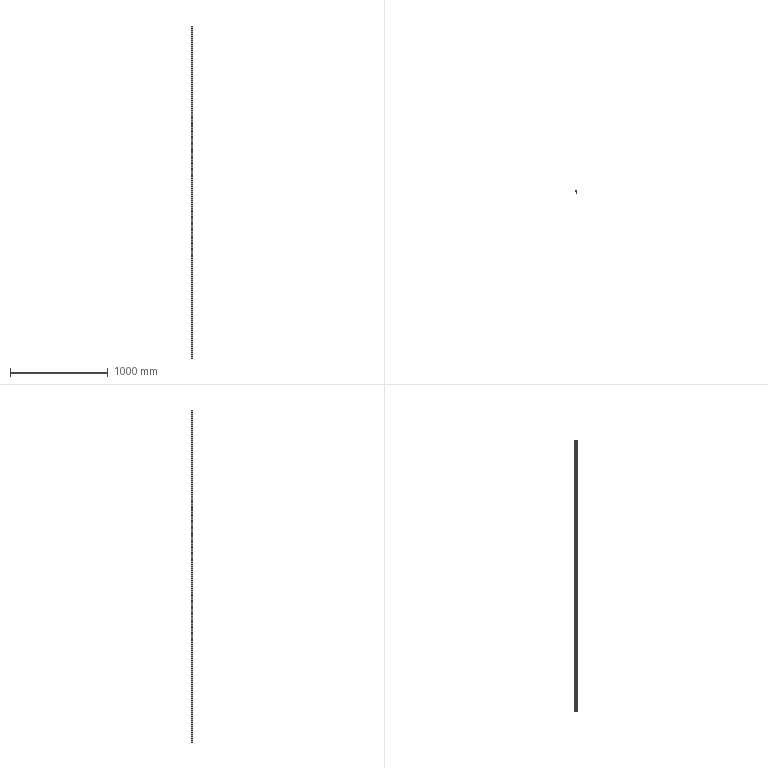Component | NX | RIB_STRIP_10 | 1 solid | 10 faces | box 14 x 15 x 3390 mm | volume 304388 mm3 | plane 10
STEP:
#1=CARTESIAN_POINT('',(0.,0.,0.));
#2=DIRECTION('',(0.,0.,1.));
#3=DIRECTION('',(1.,0.,0.));
#4=AXIS2_PLACEMENT_3D('',#1,#2,#3);
#5=CARTESIAN_POINT('',(6068.006,4310.094,-3362.));
#6=VERTEX_POINT('',#5);
#7=CARTESIAN_POINT('',(6068.006,4307.094,-3362.));
#8=VERTEX_POINT('',#7);
#9=CARTESIAN_POINT('',(6068.006,4310.094,-3362.));
#10=DIRECTION('',(0.,-1.,0.));
#11=VECTOR('',#10,1.);
#12=LINE('',#9,#11);
#13=CARTESIAN_POINT('',(6068.006,4310.094,28.));
#14=DIRECTION('',(1.,0.,0.));
#15=DIRECTION('',(0.,0.,-1.));
#16=AXIS2_PLACEMENT_3D('',#13,#14,#15);
#17=PLANE('',#16);
#18=CARTESIAN_POINT('',(3390.,0.));
#19=DIRECTION('',(0.,-1.));
#20=VECTOR('',#19,1.);
#21=LINE('',#18,#20);
#22=(GEOMETRIC_REPRESENTATION_CONTEXT(2)PARAMETRIC_REPRESENTATION_CONTEXT()REPRESENTATION_CONTEXT('',''));
#23=DEFINITIONAL_REPRESENTATION('',(#21),#22);
#24=PCURVE('',#17,#23);
#25=CARTESIAN_POINT('',(6068.006,4310.094,-3362.));
#26=DIRECTION('',(0.,0.,1.));
#27=DIRECTION('',(1.,0.,0.));
#28=AXIS2_PLACEMENT_3D('',#25,#26,#27);
#29=PLANE('',#28);
#30=CARTESIAN_POINT('',(0.,0.));
#31=DIRECTION('',(0.,-1.));
#32=VECTOR('',#31,1.);
#33=LINE('',#30,#32);
#34=(GEOMETRIC_REPRESENTATION_CONTEXT(2)PARAMETRIC_REPRESENTATION_CONTEXT()REPRESENTATION_CONTEXT('',''));
#35=DEFINITIONAL_REPRESENTATION('',(#33),#34);
#36=PCURVE('',#29,#35);
#37=SURFACE_CURVE('',#12,(#24,#36),.PCURVE_S1.);
#38=EDGE_CURVE('',#6,#8,#37,.T.);
#39=ORIENTED_EDGE('',*,*,#38,.T.);
#40=CARTESIAN_POINT('',(6068.006,4307.094,28.));
#41=VERTEX_POINT('',#40);
#42=CARTESIAN_POINT('',(6068.006,4307.094,28.));
#43=DIRECTION('',(0.,0.,-1.));
#44=VECTOR('',#43,1.);
#45=LINE('',#42,#44);
#46=CARTESIAN_POINT('',(0.,-3.));
#47=DIRECTION('',(1.,0.));
#48=VECTOR('',#47,1.);
#49=LINE('',#46,#48);
#50=(GEOMETRIC_REPRESENTATION_CONTEXT(2)PARAMETRIC_REPRESENTATION_CONTEXT()REPRESENTATION_CONTEXT('',''));
#51=DEFINITIONAL_REPRESENTATION('',(#49),#50);
#52=PCURVE('',#17,#51);
#53=CARTESIAN_POINT('',(6068.006,4307.094,28.));
#54=DIRECTION('',(0.,1.,0.));
#55=DIRECTION('',(0.,0.,1.));
#56=AXIS2_PLACEMENT_3D('',#53,#54,#55);
#57=PLANE('',#56);
#58=CARTESIAN_POINT('',(0.,0.));
#59=DIRECTION('',(-1.,0.));
#60=VECTOR('',#59,1.);
#61=LINE('',#58,#60);
#62=(GEOMETRIC_REPRESENTATION_CONTEXT(2)PARAMETRIC_REPRESENTATION_CONTEXT()REPRESENTATION_CONTEXT('',''));
#63=DEFINITIONAL_REPRESENTATION('',(#61),#62);
#64=PCURVE('',#57,#63);
#65=SURFACE_CURVE('',#45,(#52,#64),.PCURVE_S1.);
#66=EDGE_CURVE('',#41,#8,#65,.T.);
#67=ORIENTED_EDGE('',*,*,#66,.F.);
#68=CARTESIAN_POINT('',(6068.006,4310.094,28.));
#69=VERTEX_POINT('',#68);
#70=CARTESIAN_POINT('',(6068.006,4310.094,28.));
#71=DIRECTION('',(0.,-1.,0.));
#72=VECTOR('',#71,1.);
#73=LINE('',#70,#72);
#74=CARTESIAN_POINT('',(0.,0.));
#75=DIRECTION('',(0.,-1.));
#76=VECTOR('',#75,1.);
#77=LINE('',#74,#76);
#78=(GEOMETRIC_REPRESENTATION_CONTEXT(2)PARAMETRIC_REPRESENTATION_CONTEXT()REPRESENTATION_CONTEXT('',''));
#79=DEFINITIONAL_REPRESENTATION('',(#77),#78);
#80=PCURVE('',#17,#79);
#81=CARTESIAN_POINT('',(6068.006,4310.094,28.));
#82=DIRECTION('',(0.,0.,1.));
#83=DIRECTION('',(1.,0.,0.));
#84=AXIS2_PLACEMENT_3D('',#81,#82,#83);
#85=PLANE('',#84);
#86=CARTESIAN_POINT('',(0.,0.));
#87=DIRECTION('',(0.,-1.));
#88=VECTOR('',#87,1.);
#89=LINE('',#86,#88);
#90=(GEOMETRIC_REPRESENTATION_CONTEXT(2)PARAMETRIC_REPRESENTATION_CONTEXT()REPRESENTATION_CONTEXT('',''));
#91=DEFINITIONAL_REPRESENTATION('',(#89),#90);
#92=PCURVE('',#85,#91);
#93=SURFACE_CURVE('',#73,(#80,#92),.PCURVE_S1.);
#94=EDGE_CURVE('',#69,#41,#93,.T.);
#95=ORIENTED_EDGE('',*,*,#94,.F.);
#96=CARTESIAN_POINT('',(6068.006,4310.094,28.));
#97=DIRECTION('',(0.,0.,-1.));
#98=VECTOR('',#97,1.);
#99=LINE('',#96,#98);
#100=CARTESIAN_POINT('',(0.,0.));
#101=DIRECTION('',(1.,0.));
#102=VECTOR('',#101,1.);
#103=LINE('',#100,#102);
#104=(GEOMETRIC_REPRESENTATION_CONTEXT(2)PARAMETRIC_REPRESENTATION_CONTEXT()REPRESENTATION_CONTEXT('',''));
#105=DEFINITIONAL_REPRESENTATION('',(#103),#104);
#106=PCURVE('',#17,#105);
#107=CARTESIAN_POINT('',(6082.006,4310.094,28.));
#108=DIRECTION('',(0.,-1.,0.));
#109=DIRECTION('',(0.,0.,-1.));
#110=AXIS2_PLACEMENT_3D('',#107,#108,#109);
#111=PLANE('',#110);
#112=CARTESIAN_POINT('',(0.,-14.));
#113=DIRECTION('',(1.,0.));
#114=VECTOR('',#113,1.);
#115=LINE('',#112,#114);
#116=(GEOMETRIC_REPRESENTATION_CONTEXT(2)PARAMETRIC_REPRESENTATION_CONTEXT()REPRESENTATION_CONTEXT('',''));
#117=DEFINITIONAL_REPRESENTATION('',(#115),#116);
#118=PCURVE('',#111,#117);
#119=SURFACE_CURVE('',#99,(#106,#118),.PCURVE_S1.);
#120=EDGE_CURVE('',#69,#6,#119,.T.);
#121=ORIENTED_EDGE('',*,*,#120,.T.);
#122=EDGE_LOOP('',(#39,#67,#95,#121));
#123=FACE_BOUND('',#122,.T.);
#124=ADVANCED_FACE('',(#123),#17,.F.);
#125=CARTESIAN_POINT('',(6079.006,4307.094,-3362.));
#126=VERTEX_POINT('',#125);
#127=CARTESIAN_POINT('',(6068.006,4307.094,-3362.));
#128=DIRECTION('',(1.,0.,0.));
#129=VECTOR('',#128,1.);
#130=LINE('',#127,#129);
#131=CARTESIAN_POINT('',(-3390.,0.));
#132=DIRECTION('',(0.,1.));
#133=VECTOR('',#132,1.);
#134=LINE('',#131,#133);
#135=(GEOMETRIC_REPRESENTATION_CONTEXT(2)PARAMETRIC_REPRESENTATION_CONTEXT()REPRESENTATION_CONTEXT('',''));
#136=DEFINITIONAL_REPRESENTATION('',(#134),#135);
#137=PCURVE('',#57,#136);
#138=CARTESIAN_POINT('',(0.,-3.));
#139=DIRECTION('',(1.,0.));
#140=VECTOR('',#139,1.);
#141=LINE('',#138,#140);
#142=(GEOMETRIC_REPRESENTATION_CONTEXT(2)PARAMETRIC_REPRESENTATION_CONTEXT()REPRESENTATION_CONTEXT('',''));
#143=DEFINITIONAL_REPRESENTATION('',(#141),#142);
#144=PCURVE('',#29,#143);
#145=SURFACE_CURVE('',#130,(#137,#144),.PCURVE_S1.);
#146=EDGE_CURVE('',#8,#126,#145,.T.);
#147=ORIENTED_EDGE('',*,*,#146,.T.);
#148=CARTESIAN_POINT('',(6079.006,4307.094,28.));
#149=VERTEX_POINT('',#148);
#150=CARTESIAN_POINT('',(6079.006,4307.094,28.));
#151=DIRECTION('',(0.,0.,-1.));
#152=VECTOR('',#151,1.);
#153=LINE('',#150,#152);
#154=CARTESIAN_POINT('',(0.,11.));
#155=DIRECTION('',(-1.,0.));
#156=VECTOR('',#155,1.);
#157=LINE('',#154,#156);
#158=(GEOMETRIC_REPRESENTATION_CONTEXT(2)PARAMETRIC_REPRESENTATION_CONTEXT()REPRESENTATION_CONTEXT('',''));
#159=DEFINITIONAL_REPRESENTATION('',(#157),#158);
#160=PCURVE('',#57,#159);
#161=CARTESIAN_POINT('',(6079.006,4307.094,28.));
#162=DIRECTION('',(1.,0.,0.));
#163=DIRECTION('',(0.,0.,-1.));
#164=AXIS2_PLACEMENT_3D('',#161,#162,#163);
#165=PLANE('',#164);
#166=CARTESIAN_POINT('',(0.,0.));
#167=DIRECTION('',(1.,0.));
#168=VECTOR('',#167,1.);
#169=LINE('',#166,#168);
#170=(GEOMETRIC_REPRESENTATION_CONTEXT(2)PARAMETRIC_REPRESENTATION_CONTEXT()REPRESENTATION_CONTEXT('',''));
#171=DEFINITIONAL_REPRESENTATION('',(#169),#170);
#172=PCURVE('',#165,#171);
#173=SURFACE_CURVE('',#153,(#160,#172),.PCURVE_S1.);
#174=EDGE_CURVE('',#149,#126,#173,.T.);
#175=ORIENTED_EDGE('',*,*,#174,.F.);
#176=CARTESIAN_POINT('',(6068.006,4307.094,28.));
#177=DIRECTION('',(1.,0.,0.));
#178=VECTOR('',#177,1.);
#179=LINE('',#176,#178);
#180=CARTESIAN_POINT('',(0.,0.));
#181=DIRECTION('',(0.,1.));
#182=VECTOR('',#181,1.);
#183=LINE('',#180,#182);
#184=(GEOMETRIC_REPRESENTATION_CONTEXT(2)PARAMETRIC_REPRESENTATION_CONTEXT()REPRESENTATION_CONTEXT('',''));
#185=DEFINITIONAL_REPRESENTATION('',(#183),#184);
#186=PCURVE('',#57,#185);
#187=CARTESIAN_POINT('',(0.,-3.));
#188=DIRECTION('',(1.,0.));
#189=VECTOR('',#188,1.);
#190=LINE('',#187,#189);
#191=(GEOMETRIC_REPRESENTATION_CONTEXT(2)PARAMETRIC_REPRESENTATION_CONTEXT()REPRESENTATION_CONTEXT('',''));
#192=DEFINITIONAL_REPRESENTATION('',(#190),#191);
#193=PCURVE('',#85,#192);
#194=SURFACE_CURVE('',#179,(#186,#193),.PCURVE_S1.);
#195=EDGE_CURVE('',#41,#149,#194,.T.);
#196=ORIENTED_EDGE('',*,*,#195,.F.);
#197=ORIENTED_EDGE('',*,*,#66,.T.);
#198=EDGE_LOOP('',(#147,#175,#196,#197));
#199=FACE_BOUND('',#198,.T.);
#200=ADVANCED_FACE('',(#199),#57,.F.);
#201=CARTESIAN_POINT('',(6079.006,4298.042,-3362.));
#202=VERTEX_POINT('',#201);
#203=CARTESIAN_POINT('',(6079.006,4307.094,-3362.));
#204=DIRECTION('',(0.,-1.,0.));
#205=VECTOR('',#204,1.);
#206=LINE('',#203,#205);
#207=CARTESIAN_POINT('',(3390.,0.));
#208=DIRECTION('',(0.,-1.));
#209=VECTOR('',#208,1.);
#210=LINE('',#207,#209);
#211=(GEOMETRIC_REPRESENTATION_CONTEXT(2)PARAMETRIC_REPRESENTATION_CONTEXT()REPRESENTATION_CONTEXT('',''));
#212=DEFINITIONAL_REPRESENTATION('',(#210),#211);
#213=PCURVE('',#165,#212);
#214=CARTESIAN_POINT('',(11.,-3.));
#215=DIRECTION('',(0.,-1.));
#216=VECTOR('',#215,1.);
#217=LINE('',#214,#216);
#218=(GEOMETRIC_REPRESENTATION_CONTEXT(2)PARAMETRIC_REPRESENTATION_CONTEXT()REPRESENTATION_CONTEXT('',''));
#219=DEFINITIONAL_REPRESENTATION('',(#217),#218);
#220=PCURVE('',#29,#219);
#221=SURFACE_CURVE('',#206,(#213,#220),.PCURVE_S1.);
#222=EDGE_CURVE('',#126,#202,#221,.T.);
#223=ORIENTED_EDGE('',*,*,#222,.T.);
#224=CARTESIAN_POINT('',(6079.006,4298.042,28.));
#225=VERTEX_POINT('',#224);
#226=CARTESIAN_POINT('',(6079.006,4298.042,28.));
#227=DIRECTION('',(0.,0.,-1.));
#228=VECTOR('',#227,1.);
#229=LINE('',#226,#228);
#230=CARTESIAN_POINT('',(0.,-9.052));
#231=DIRECTION('',(1.,0.));
#232=VECTOR('',#231,1.);
#233=LINE('',#230,#232);
#234=(GEOMETRIC_REPRESENTATION_CONTEXT(2)PARAMETRIC_REPRESENTATION_CONTEXT()REPRESENTATION_CONTEXT('',''));
#235=DEFINITIONAL_REPRESENTATION('',(#233),#234);
#236=PCURVE('',#165,#235);
#237=CARTESIAN_POINT('',(6079.006,4298.042,28.));
#238=DIRECTION('',(0.,-1.,0.));
#239=DIRECTION('',(0.,0.,-1.));
#240=AXIS2_PLACEMENT_3D('',#237,#238,#239);
#241=PLANE('',#240);
#242=CARTESIAN_POINT('',(0.,0.));
#243=DIRECTION('',(1.,0.));
#244=VECTOR('',#243,1.);
#245=LINE('',#242,#244);
#246=(GEOMETRIC_REPRESENTATION_CONTEXT(2)PARAMETRIC_REPRESENTATION_CONTEXT()REPRESENTATION_CONTEXT('',''));
#247=DEFINITIONAL_REPRESENTATION('',(#245),#246);
#248=PCURVE('',#241,#247);
#249=SURFACE_CURVE('',#229,(#236,#248),.PCURVE_S1.);
#250=EDGE_CURVE('',#225,#202,#249,.T.);
#251=ORIENTED_EDGE('',*,*,#250,.F.);
#252=CARTESIAN_POINT('',(6079.006,4307.094,28.));
#253=DIRECTION('',(0.,-1.,0.));
#254=VECTOR('',#253,1.);
#255=LINE('',#252,#254);
#256=CARTESIAN_POINT('',(0.,0.));
#257=DIRECTION('',(0.,-1.));
#258=VECTOR('',#257,1.);
#259=LINE('',#256,#258);
#260=(GEOMETRIC_REPRESENTATION_CONTEXT(2)PARAMETRIC_REPRESENTATION_CONTEXT()REPRESENTATION_CONTEXT('',''));
#261=DEFINITIONAL_REPRESENTATION('',(#259),#260);
#262=PCURVE('',#165,#261);
#263=CARTESIAN_POINT('',(11.,-3.));
#264=DIRECTION('',(0.,-1.));
#265=VECTOR('',#264,1.);
#266=LINE('',#263,#265);
#267=(GEOMETRIC_REPRESENTATION_CONTEXT(2)PARAMETRIC_REPRESENTATION_CONTEXT()REPRESENTATION_CONTEXT('',''));
#268=DEFINITIONAL_REPRESENTATION('',(#266),#267);
#269=PCURVE('',#85,#268);
#270=SURFACE_CURVE('',#255,(#262,#269),.PCURVE_S1.);
#271=EDGE_CURVE('',#149,#225,#270,.T.);
#272=ORIENTED_EDGE('',*,*,#271,.F.);
#273=ORIENTED_EDGE('',*,*,#174,.T.);
#274=EDGE_LOOP('',(#223,#251,#272,#273));
#275=FACE_BOUND('',#274,.T.);
#276=ADVANCED_FACE('',(#275),#165,.F.);
#277=CARTESIAN_POINT('',(6075.006,4298.042,-3362.));
#278=VERTEX_POINT('',#277);
#279=CARTESIAN_POINT('',(6079.006,4298.042,-3362.));
#280=DIRECTION('',(-1.,0.,0.));
#281=VECTOR('',#280,1.);
#282=LINE('',#279,#281);
#283=CARTESIAN_POINT('',(3390.,0.));
#284=DIRECTION('',(0.,-1.));
#285=VECTOR('',#284,1.);
#286=LINE('',#283,#285);
#287=(GEOMETRIC_REPRESENTATION_CONTEXT(2)PARAMETRIC_REPRESENTATION_CONTEXT()REPRESENTATION_CONTEXT('',''));
#288=DEFINITIONAL_REPRESENTATION('',(#286),#287);
#289=PCURVE('',#241,#288);
#290=CARTESIAN_POINT('',(11.,-12.052));
#291=DIRECTION('',(-1.,0.));
#292=VECTOR('',#291,1.);
#293=LINE('',#290,#292);
#294=(GEOMETRIC_REPRESENTATION_CONTEXT(2)PARAMETRIC_REPRESENTATION_CONTEXT()REPRESENTATION_CONTEXT('',''));
#295=DEFINITIONAL_REPRESENTATION('',(#293),#294);
#296=PCURVE('',#29,#295);
#297=SURFACE_CURVE('',#282,(#289,#296),.PCURVE_S1.);
#298=EDGE_CURVE('',#202,#278,#297,.T.);
#299=ORIENTED_EDGE('',*,*,#298,.T.);
#300=CARTESIAN_POINT('',(6075.006,4298.042,28.));
#301=VERTEX_POINT('',#300);
#302=CARTESIAN_POINT('',(6075.006,4298.042,28.));
#303=DIRECTION('',(0.,0.,-1.));
#304=VECTOR('',#303,1.);
#305=LINE('',#302,#304);
#306=CARTESIAN_POINT('',(0.,-4.));
#307=DIRECTION('',(1.,0.));
#308=VECTOR('',#307,1.);
#309=LINE('',#306,#308);
#310=(GEOMETRIC_REPRESENTATION_CONTEXT(2)PARAMETRIC_REPRESENTATION_CONTEXT()REPRESENTATION_CONTEXT('',''));
#311=DEFINITIONAL_REPRESENTATION('',(#309),#310);
#312=PCURVE('',#241,#311);
#313=CARTESIAN_POINT('',(6075.006,4298.042,28.));
#314=DIRECTION('',(1.,0.,0.));
#315=DIRECTION('',(0.,0.,-1.));
#316=AXIS2_PLACEMENT_3D('',#313,#314,#315);
#317=PLANE('',#316);
#318=CARTESIAN_POINT('',(0.,0.));
#319=DIRECTION('',(1.,0.));
#320=VECTOR('',#319,1.);
#321=LINE('',#318,#320);
#322=(GEOMETRIC_REPRESENTATION_CONTEXT(2)PARAMETRIC_REPRESENTATION_CONTEXT()REPRESENTATION_CONTEXT('',''));
#323=DEFINITIONAL_REPRESENTATION('',(#321),#322);
#324=PCURVE('',#317,#323);
#325=SURFACE_CURVE('',#305,(#312,#324),.PCURVE_S1.);
#326=EDGE_CURVE('',#301,#278,#325,.T.);
#327=ORIENTED_EDGE('',*,*,#326,.F.);
#328=CARTESIAN_POINT('',(6079.006,4298.042,28.));
#329=DIRECTION('',(-1.,0.,0.));
#330=VECTOR('',#329,1.);
#331=LINE('',#328,#330);
#332=CARTESIAN_POINT('',(0.,0.));
#333=DIRECTION('',(0.,-1.));
#334=VECTOR('',#333,1.);
#335=LINE('',#332,#334);
#336=(GEOMETRIC_REPRESENTATION_CONTEXT(2)PARAMETRIC_REPRESENTATION_CONTEXT()REPRESENTATION_CONTEXT('',''));
#337=DEFINITIONAL_REPRESENTATION('',(#335),#336);
#338=PCURVE('',#241,#337);
#339=CARTESIAN_POINT('',(11.,-12.052));
#340=DIRECTION('',(-1.,0.));
#341=VECTOR('',#340,1.);
#342=LINE('',#339,#341);
#343=(GEOMETRIC_REPRESENTATION_CONTEXT(2)PARAMETRIC_REPRESENTATION_CONTEXT()REPRESENTATION_CONTEXT('',''));
#344=DEFINITIONAL_REPRESENTATION('',(#342),#343);
#345=PCURVE('',#85,#344);
#346=SURFACE_CURVE('',#331,(#338,#345),.PCURVE_S1.);
#347=EDGE_CURVE('',#225,#301,#346,.T.);
#348=ORIENTED_EDGE('',*,*,#347,.F.);
#349=ORIENTED_EDGE('',*,*,#250,.T.);
#350=EDGE_LOOP('',(#299,#327,#348,#349));
#351=FACE_BOUND('',#350,.T.);
#352=ADVANCED_FACE('',(#351),#241,.F.);
#353=CARTESIAN_POINT('',(6075.006,4295.094,-3362.));
#354=VERTEX_POINT('',#353);
#355=CARTESIAN_POINT('',(6075.006,4298.042,-3362.));
#356=DIRECTION('',(0.,-1.,0.));
#357=VECTOR('',#356,1.);
#358=LINE('',#355,#357);
#359=CARTESIAN_POINT('',(3390.,0.));
#360=DIRECTION('',(0.,-1.));
#361=VECTOR('',#360,1.);
#362=LINE('',#359,#361);
#363=(GEOMETRIC_REPRESENTATION_CONTEXT(2)PARAMETRIC_REPRESENTATION_CONTEXT()REPRESENTATION_CONTEXT('',''));
#364=DEFINITIONAL_REPRESENTATION('',(#362),#363);
#365=PCURVE('',#317,#364);
#366=CARTESIAN_POINT('',(7.,-12.052));
#367=DIRECTION('',(0.,-1.));
#368=VECTOR('',#367,1.);
#369=LINE('',#366,#368);
#370=(GEOMETRIC_REPRESENTATION_CONTEXT(2)PARAMETRIC_REPRESENTATION_CONTEXT()REPRESENTATION_CONTEXT('',''));
#371=DEFINITIONAL_REPRESENTATION('',(#369),#370);
#372=PCURVE('',#29,#371);
#373=SURFACE_CURVE('',#358,(#365,#372),.PCURVE_S1.);
#374=EDGE_CURVE('',#278,#354,#373,.T.);
#375=ORIENTED_EDGE('',*,*,#374,.T.);
#376=CARTESIAN_POINT('',(6075.006,4295.094,28.));
#377=VERTEX_POINT('',#376);
#378=CARTESIAN_POINT('',(6075.006,4295.094,28.));
#379=DIRECTION('',(0.,0.,-1.));
#380=VECTOR('',#379,1.);
#381=LINE('',#378,#380);
#382=CARTESIAN_POINT('',(0.,-2.948));
#383=DIRECTION('',(1.,0.));
#384=VECTOR('',#383,1.);
#385=LINE('',#382,#384);
#386=(GEOMETRIC_REPRESENTATION_CONTEXT(2)PARAMETRIC_REPRESENTATION_CONTEXT()REPRESENTATION_CONTEXT('',''));
#387=DEFINITIONAL_REPRESENTATION('',(#385),#386);
#388=PCURVE('',#317,#387);
#389=CARTESIAN_POINT('',(6075.006,4295.094,28.));
#390=DIRECTION('',(0.,1.,0.));
#391=DIRECTION('',(0.,0.,1.));
#392=AXIS2_PLACEMENT_3D('',#389,#390,#391);
#393=PLANE('',#392);
#394=CARTESIAN_POINT('',(0.,0.));
#395=DIRECTION('',(-1.,0.));
#396=VECTOR('',#395,1.);
#397=LINE('',#394,#396);
#398=(GEOMETRIC_REPRESENTATION_CONTEXT(2)PARAMETRIC_REPRESENTATION_CONTEXT()REPRESENTATION_CONTEXT('',''));
#399=DEFINITIONAL_REPRESENTATION('',(#397),#398);
#400=PCURVE('',#393,#399);
#401=SURFACE_CURVE('',#381,(#388,#400),.PCURVE_S1.);
#402=EDGE_CURVE('',#377,#354,#401,.T.);
#403=ORIENTED_EDGE('',*,*,#402,.F.);
#404=CARTESIAN_POINT('',(6075.006,4298.042,28.));
#405=DIRECTION('',(0.,-1.,0.));
#406=VECTOR('',#405,1.);
#407=LINE('',#404,#406);
#408=CARTESIAN_POINT('',(0.,0.));
#409=DIRECTION('',(0.,-1.));
#410=VECTOR('',#409,1.);
#411=LINE('',#408,#410);
#412=(GEOMETRIC_REPRESENTATION_CONTEXT(2)PARAMETRIC_REPRESENTATION_CONTEXT()REPRESENTATION_CONTEXT('',''));
#413=DEFINITIONAL_REPRESENTATION('',(#411),#412);
#414=PCURVE('',#317,#413);
#415=CARTESIAN_POINT('',(7.,-12.052));
#416=DIRECTION('',(0.,-1.));
#417=VECTOR('',#416,1.);
#418=LINE('',#415,#417);
#419=(GEOMETRIC_REPRESENTATION_CONTEXT(2)PARAMETRIC_REPRESENTATION_CONTEXT()REPRESENTATION_CONTEXT('',''));
#420=DEFINITIONAL_REPRESENTATION('',(#418),#419);
#421=PCURVE('',#85,#420);
#422=SURFACE_CURVE('',#407,(#414,#421),.PCURVE_S1.);
#423=EDGE_CURVE('',#301,#377,#422,.T.);
#424=ORIENTED_EDGE('',*,*,#423,.F.);
#425=ORIENTED_EDGE('',*,*,#326,.T.);
#426=EDGE_LOOP('',(#375,#403,#424,#425));
#427=FACE_BOUND('',#426,.T.);
#428=ADVANCED_FACE('',(#427),#317,.F.);
#429=CARTESIAN_POINT('',(6082.006,4295.094,-3362.));
#430=VERTEX_POINT('',#429);
#431=CARTESIAN_POINT('',(6075.006,4295.094,-3362.));
#432=DIRECTION('',(1.,0.,0.));
#433=VECTOR('',#432,1.);
#434=LINE('',#431,#433);
#435=CARTESIAN_POINT('',(-3390.,0.));
#436=DIRECTION('',(0.,1.));
#437=VECTOR('',#436,1.);
#438=LINE('',#435,#437);
#439=(GEOMETRIC_REPRESENTATION_CONTEXT(2)PARAMETRIC_REPRESENTATION_CONTEXT()REPRESENTATION_CONTEXT('',''));
#440=DEFINITIONAL_REPRESENTATION('',(#438),#439);
#441=PCURVE('',#393,#440);
#442=CARTESIAN_POINT('',(7.,-15.));
#443=DIRECTION('',(1.,0.));
#444=VECTOR('',#443,1.);
#445=LINE('',#442,#444);
#446=(GEOMETRIC_REPRESENTATION_CONTEXT(2)PARAMETRIC_REPRESENTATION_CONTEXT()REPRESENTATION_CONTEXT('',''));
#447=DEFINITIONAL_REPRESENTATION('',(#445),#446);
#448=PCURVE('',#29,#447);
#449=SURFACE_CURVE('',#434,(#441,#448),.PCURVE_S1.);
#450=EDGE_CURVE('',#354,#430,#449,.T.);
#451=ORIENTED_EDGE('',*,*,#450,.T.);
#452=CARTESIAN_POINT('',(6082.006,4295.094,28.));
#453=VERTEX_POINT('',#452);
#454=CARTESIAN_POINT('',(6082.006,4295.094,28.));
#455=DIRECTION('',(0.,0.,-1.));
#456=VECTOR('',#455,1.);
#457=LINE('',#454,#456);
#458=CARTESIAN_POINT('',(0.,7.));
#459=DIRECTION('',(-1.,0.));
#460=VECTOR('',#459,1.);
#461=LINE('',#458,#460);
#462=(GEOMETRIC_REPRESENTATION_CONTEXT(2)PARAMETRIC_REPRESENTATION_CONTEXT()REPRESENTATION_CONTEXT('',''));
#463=DEFINITIONAL_REPRESENTATION('',(#461),#462);
#464=PCURVE('',#393,#463);
#465=CARTESIAN_POINT('',(6082.006,4295.094,28.));
#466=DIRECTION('',(-1.,0.,0.));
#467=DIRECTION('',(0.,0.,1.));
#468=AXIS2_PLACEMENT_3D('',#465,#466,#467);
#469=PLANE('',#468);
#470=CARTESIAN_POINT('',(0.,0.));
#471=DIRECTION('',(-1.,0.));
#472=VECTOR('',#471,1.);
#473=LINE('',#470,#472);
#474=(GEOMETRIC_REPRESENTATION_CONTEXT(2)PARAMETRIC_REPRESENTATION_CONTEXT()REPRESENTATION_CONTEXT('',''));
#475=DEFINITIONAL_REPRESENTATION('',(#473),#474);
#476=PCURVE('',#469,#475);
#477=SURFACE_CURVE('',#457,(#464,#476),.PCURVE_S1.);
#478=EDGE_CURVE('',#453,#430,#477,.T.);
#479=ORIENTED_EDGE('',*,*,#478,.F.);
#480=CARTESIAN_POINT('',(6075.006,4295.094,28.));
#481=DIRECTION('',(1.,0.,0.));
#482=VECTOR('',#481,1.);
#483=LINE('',#480,#482);
#484=CARTESIAN_POINT('',(0.,0.));
#485=DIRECTION('',(0.,1.));
#486=VECTOR('',#485,1.);
#487=LINE('',#484,#486);
#488=(GEOMETRIC_REPRESENTATION_CONTEXT(2)PARAMETRIC_REPRESENTATION_CONTEXT()REPRESENTATION_CONTEXT('',''));
#489=DEFINITIONAL_REPRESENTATION('',(#487),#488);
#490=PCURVE('',#393,#489);
#491=CARTESIAN_POINT('',(7.,-15.));
#492=DIRECTION('',(1.,0.));
#493=VECTOR('',#492,1.);
#494=LINE('',#491,#493);
#495=(GEOMETRIC_REPRESENTATION_CONTEXT(2)PARAMETRIC_REPRESENTATION_CONTEXT()REPRESENTATION_CONTEXT('',''));
#496=DEFINITIONAL_REPRESENTATION('',(#494),#495);
#497=PCURVE('',#85,#496);
#498=SURFACE_CURVE('',#483,(#490,#497),.PCURVE_S1.);
#499=EDGE_CURVE('',#377,#453,#498,.T.);
#500=ORIENTED_EDGE('',*,*,#499,.F.);
#501=ORIENTED_EDGE('',*,*,#402,.T.);
#502=EDGE_LOOP('',(#451,#479,#500,#501));
#503=FACE_BOUND('',#502,.T.);
#504=ADVANCED_FACE('',(#503),#393,.F.);
#505=CARTESIAN_POINT('',(6082.006,4310.094,-3362.));
#506=VERTEX_POINT('',#505);
#507=CARTESIAN_POINT('',(6082.006,4295.094,-3362.));
#508=DIRECTION('',(0.,1.,0.));
#509=VECTOR('',#508,1.);
#510=LINE('',#507,#509);
#511=CARTESIAN_POINT('',(-3390.,0.));
#512=DIRECTION('',(0.,1.));
#513=VECTOR('',#512,1.);
#514=LINE('',#511,#513);
#515=(GEOMETRIC_REPRESENTATION_CONTEXT(2)PARAMETRIC_REPRESENTATION_CONTEXT()REPRESENTATION_CONTEXT('',''));
#516=DEFINITIONAL_REPRESENTATION('',(#514),#515);
#517=PCURVE('',#469,#516);
#518=CARTESIAN_POINT('',(14.,-15.));
#519=DIRECTION('',(0.,1.));
#520=VECTOR('',#519,1.);
#521=LINE('',#518,#520);
#522=(GEOMETRIC_REPRESENTATION_CONTEXT(2)PARAMETRIC_REPRESENTATION_CONTEXT()REPRESENTATION_CONTEXT('',''));
#523=DEFINITIONAL_REPRESENTATION('',(#521),#522);
#524=PCURVE('',#29,#523);
#525=SURFACE_CURVE('',#510,(#517,#524),.PCURVE_S1.);
#526=EDGE_CURVE('',#430,#506,#525,.T.);
#527=ORIENTED_EDGE('',*,*,#526,.T.);
#528=CARTESIAN_POINT('',(6082.006,4310.094,28.));
#529=VERTEX_POINT('',#528);
#530=CARTESIAN_POINT('',(6082.006,4310.094,28.));
#531=DIRECTION('',(0.,0.,-1.));
#532=VECTOR('',#531,1.);
#533=LINE('',#530,#532);
#534=CARTESIAN_POINT('',(0.,15.));
#535=DIRECTION('',(-1.,0.));
#536=VECTOR('',#535,1.);
#537=LINE('',#534,#536);
#538=(GEOMETRIC_REPRESENTATION_CONTEXT(2)PARAMETRIC_REPRESENTATION_CONTEXT()REPRESENTATION_CONTEXT('',''));
#539=DEFINITIONAL_REPRESENTATION('',(#537),#538);
#540=PCURVE('',#469,#539);
#541=CARTESIAN_POINT('',(0.,0.));
#542=DIRECTION('',(1.,0.));
#543=VECTOR('',#542,1.);
#544=LINE('',#541,#543);
#545=(GEOMETRIC_REPRESENTATION_CONTEXT(2)PARAMETRIC_REPRESENTATION_CONTEXT()REPRESENTATION_CONTEXT('',''));
#546=DEFINITIONAL_REPRESENTATION('',(#544),#545);
#547=PCURVE('',#111,#546);
#548=SURFACE_CURVE('',#533,(#540,#547),.PCURVE_S1.);
#549=EDGE_CURVE('',#529,#506,#548,.T.);
#550=ORIENTED_EDGE('',*,*,#549,.F.);
#551=CARTESIAN_POINT('',(6082.006,4295.094,28.));
#552=DIRECTION('',(0.,1.,0.));
#553=VECTOR('',#552,1.);
#554=LINE('',#551,#553);
#555=CARTESIAN_POINT('',(0.,0.));
#556=DIRECTION('',(0.,1.));
#557=VECTOR('',#556,1.);
#558=LINE('',#555,#557);
#559=(GEOMETRIC_REPRESENTATION_CONTEXT(2)PARAMETRIC_REPRESENTATION_CONTEXT()REPRESENTATION_CONTEXT('',''));
#560=DEFINITIONAL_REPRESENTATION('',(#558),#559);
#561=PCURVE('',#469,#560);
#562=CARTESIAN_POINT('',(14.,-15.));
#563=DIRECTION('',(0.,1.));
#564=VECTOR('',#563,1.);
#565=LINE('',#562,#564);
#566=(GEOMETRIC_REPRESENTATION_CONTEXT(2)PARAMETRIC_REPRESENTATION_CONTEXT()REPRESENTATION_CONTEXT('',''));
#567=DEFINITIONAL_REPRESENTATION('',(#565),#566);
#568=PCURVE('',#85,#567);
#569=SURFACE_CURVE('',#554,(#561,#568),.PCURVE_S1.);
#570=EDGE_CURVE('',#453,#529,#569,.T.);
#571=ORIENTED_EDGE('',*,*,#570,.F.);
#572=ORIENTED_EDGE('',*,*,#478,.T.);
#573=EDGE_LOOP('',(#527,#550,#571,#572));
#574=FACE_BOUND('',#573,.T.);
#575=ADVANCED_FACE('',(#574),#469,.F.);
#576=CARTESIAN_POINT('',(6082.006,4310.094,-3362.));
#577=DIRECTION('',(-1.,0.,0.));
#578=VECTOR('',#577,1.);
#579=LINE('',#576,#578);
#580=CARTESIAN_POINT('',(3390.,0.));
#581=DIRECTION('',(0.,-1.));
#582=VECTOR('',#581,1.);
#583=LINE('',#580,#582);
#584=(GEOMETRIC_REPRESENTATION_CONTEXT(2)PARAMETRIC_REPRESENTATION_CONTEXT()REPRESENTATION_CONTEXT('',''));
#585=DEFINITIONAL_REPRESENTATION('',(#583),#584);
#586=PCURVE('',#111,#585);
#587=CARTESIAN_POINT('',(14.,0.));
#588=DIRECTION('',(-1.,0.));
#589=VECTOR('',#588,1.);
#590=LINE('',#587,#589);
#591=(GEOMETRIC_REPRESENTATION_CONTEXT(2)PARAMETRIC_REPRESENTATION_CONTEXT()REPRESENTATION_CONTEXT('',''));
#592=DEFINITIONAL_REPRESENTATION('',(#590),#591);
#593=PCURVE('',#29,#592);
#594=SURFACE_CURVE('',#579,(#586,#593),.PCURVE_S1.);
#595=EDGE_CURVE('',#506,#6,#594,.T.);
#596=ORIENTED_EDGE('',*,*,#595,.T.);
#597=ORIENTED_EDGE('',*,*,#120,.F.);
#598=CARTESIAN_POINT('',(6082.006,4310.094,28.));
#599=DIRECTION('',(-1.,0.,0.));
#600=VECTOR('',#599,1.);
#601=LINE('',#598,#600);
#602=CARTESIAN_POINT('',(0.,0.));
#603=DIRECTION('',(0.,-1.));
#604=VECTOR('',#603,1.);
#605=LINE('',#602,#604);
#606=(GEOMETRIC_REPRESENTATION_CONTEXT(2)PARAMETRIC_REPRESENTATION_CONTEXT()REPRESENTATION_CONTEXT('',''));
#607=DEFINITIONAL_REPRESENTATION('',(#605),#606);
#608=PCURVE('',#111,#607);
#609=CARTESIAN_POINT('',(14.,0.));
#610=DIRECTION('',(-1.,0.));
#611=VECTOR('',#610,1.);
#612=LINE('',#609,#611);
#613=(GEOMETRIC_REPRESENTATION_CONTEXT(2)PARAMETRIC_REPRESENTATION_CONTEXT()REPRESENTATION_CONTEXT('',''));
#614=DEFINITIONAL_REPRESENTATION('',(#612),#613);
#615=PCURVE('',#85,#614);
#616=SURFACE_CURVE('',#601,(#608,#615),.PCURVE_S1.);
#617=EDGE_CURVE('',#529,#69,#616,.T.);
#618=ORIENTED_EDGE('',*,*,#617,.F.);
#619=ORIENTED_EDGE('',*,*,#549,.T.);
#620=EDGE_LOOP('',(#596,#597,#618,#619));
#621=FACE_BOUND('',#620,.T.);
#622=ADVANCED_FACE('',(#621),#111,.F.);
#623=ORIENTED_EDGE('',*,*,#94,.T.);
#624=ORIENTED_EDGE('',*,*,#195,.T.);
#625=ORIENTED_EDGE('',*,*,#271,.T.);
#626=ORIENTED_EDGE('',*,*,#347,.T.);
#627=ORIENTED_EDGE('',*,*,#423,.T.);
#628=ORIENTED_EDGE('',*,*,#499,.T.);
#629=ORIENTED_EDGE('',*,*,#570,.T.);
#630=ORIENTED_EDGE('',*,*,#617,.T.);
#631=EDGE_LOOP('',(#623,#624,#625,#626,#627,#628,#629,#630));
#632=FACE_BOUND('',#631,.T.);
#633=ADVANCED_FACE('',(#632),#85,.T.);
#634=ORIENTED_EDGE('',*,*,#38,.F.);
#635=ORIENTED_EDGE('',*,*,#595,.F.);
#636=ORIENTED_EDGE('',*,*,#526,.F.);
#637=ORIENTED_EDGE('',*,*,#450,.F.);
#638=ORIENTED_EDGE('',*,*,#374,.F.);
#639=ORIENTED_EDGE('',*,*,#298,.F.);
#640=ORIENTED_EDGE('',*,*,#222,.F.);
#641=ORIENTED_EDGE('',*,*,#146,.F.);
#642=EDGE_LOOP('',(#634,#635,#636,#637,#638,#639,#640,#641));
#643=FACE_BOUND('',#642,.T.);
#644=ADVANCED_FACE('',(#643),#29,.F.);
#645=CLOSED_SHELL('',(#124,#200,#276,#352,#428,#504,#575,#622,#633,#644));
#646=MANIFOLD_SOLID_BREP('',#645);
#647=(LENGTH_UNIT()NAMED_UNIT(*)SI_UNIT(.MILLI.,.METRE.));
#648=UNCERTAINTY_MEASURE_WITH_UNIT(LENGTH_MEASURE(0.0000001),#647,'','');
#649=(NAMED_UNIT(*)PLANE_ANGLE_UNIT()SI_UNIT($,.RADIAN.));
#650=(NAMED_UNIT(*)SI_UNIT($,.STERADIAN.)SOLID_ANGLE_UNIT());
#651=(GEOMETRIC_REPRESENTATION_CONTEXT(3)GLOBAL_UNCERTAINTY_ASSIGNED_CONTEXT((#648))GLOBAL_UNIT_ASSIGNED_CONTEXT((#647,#649,#650))REPRESENTATION_CONTEXT('',''));
#652=ADVANCED_BREP_SHAPE_REPRESENTATION('',(#4,#646),#651);